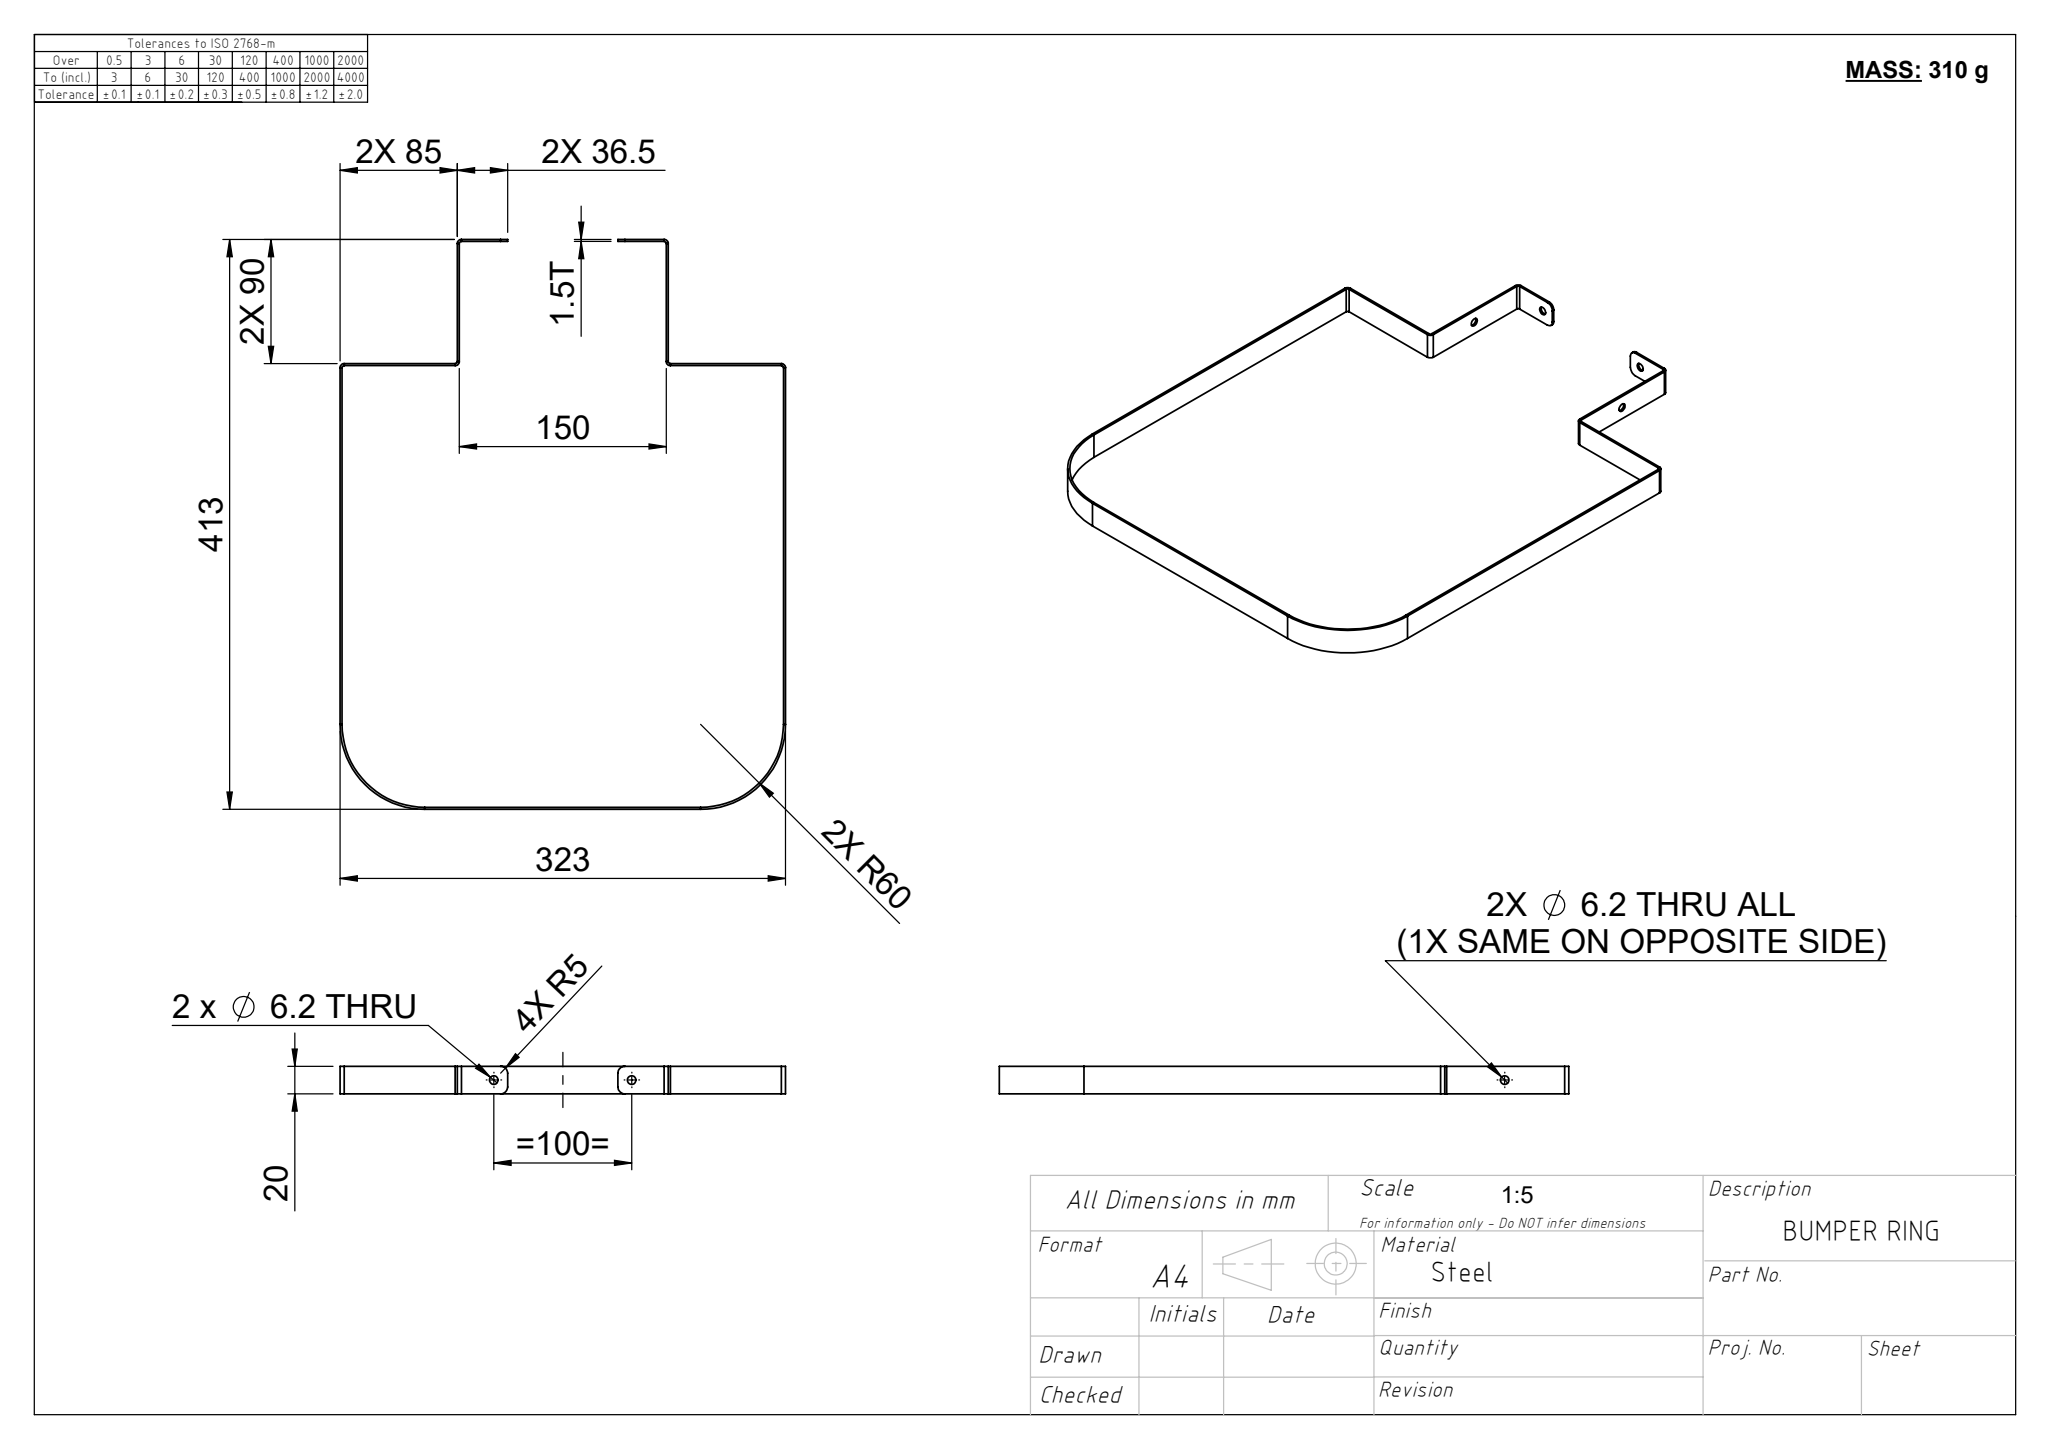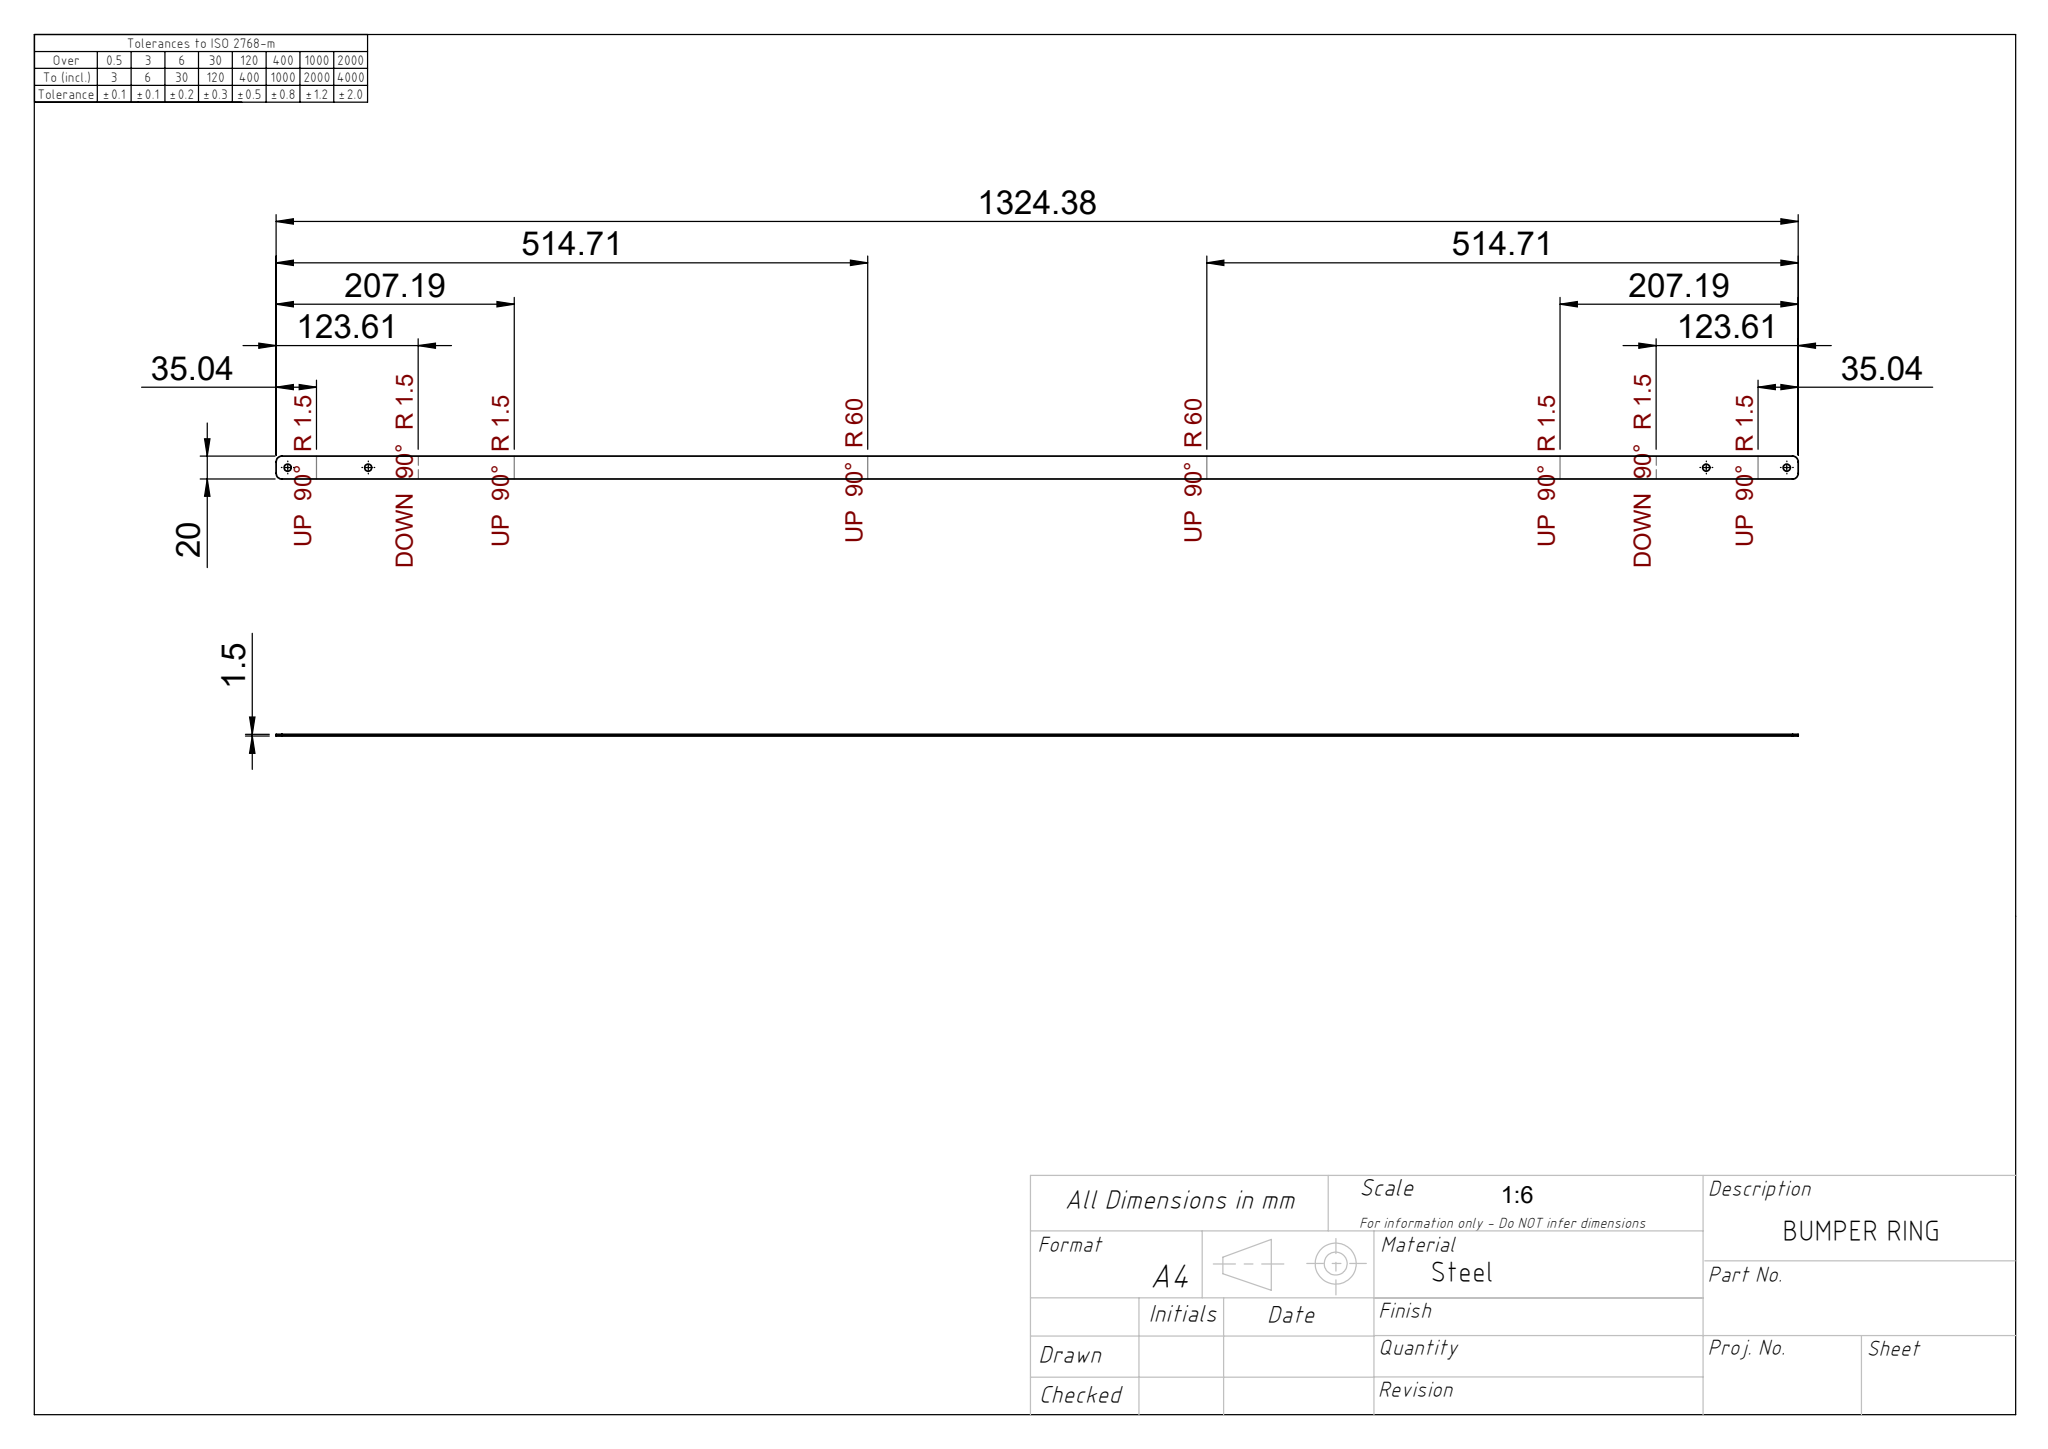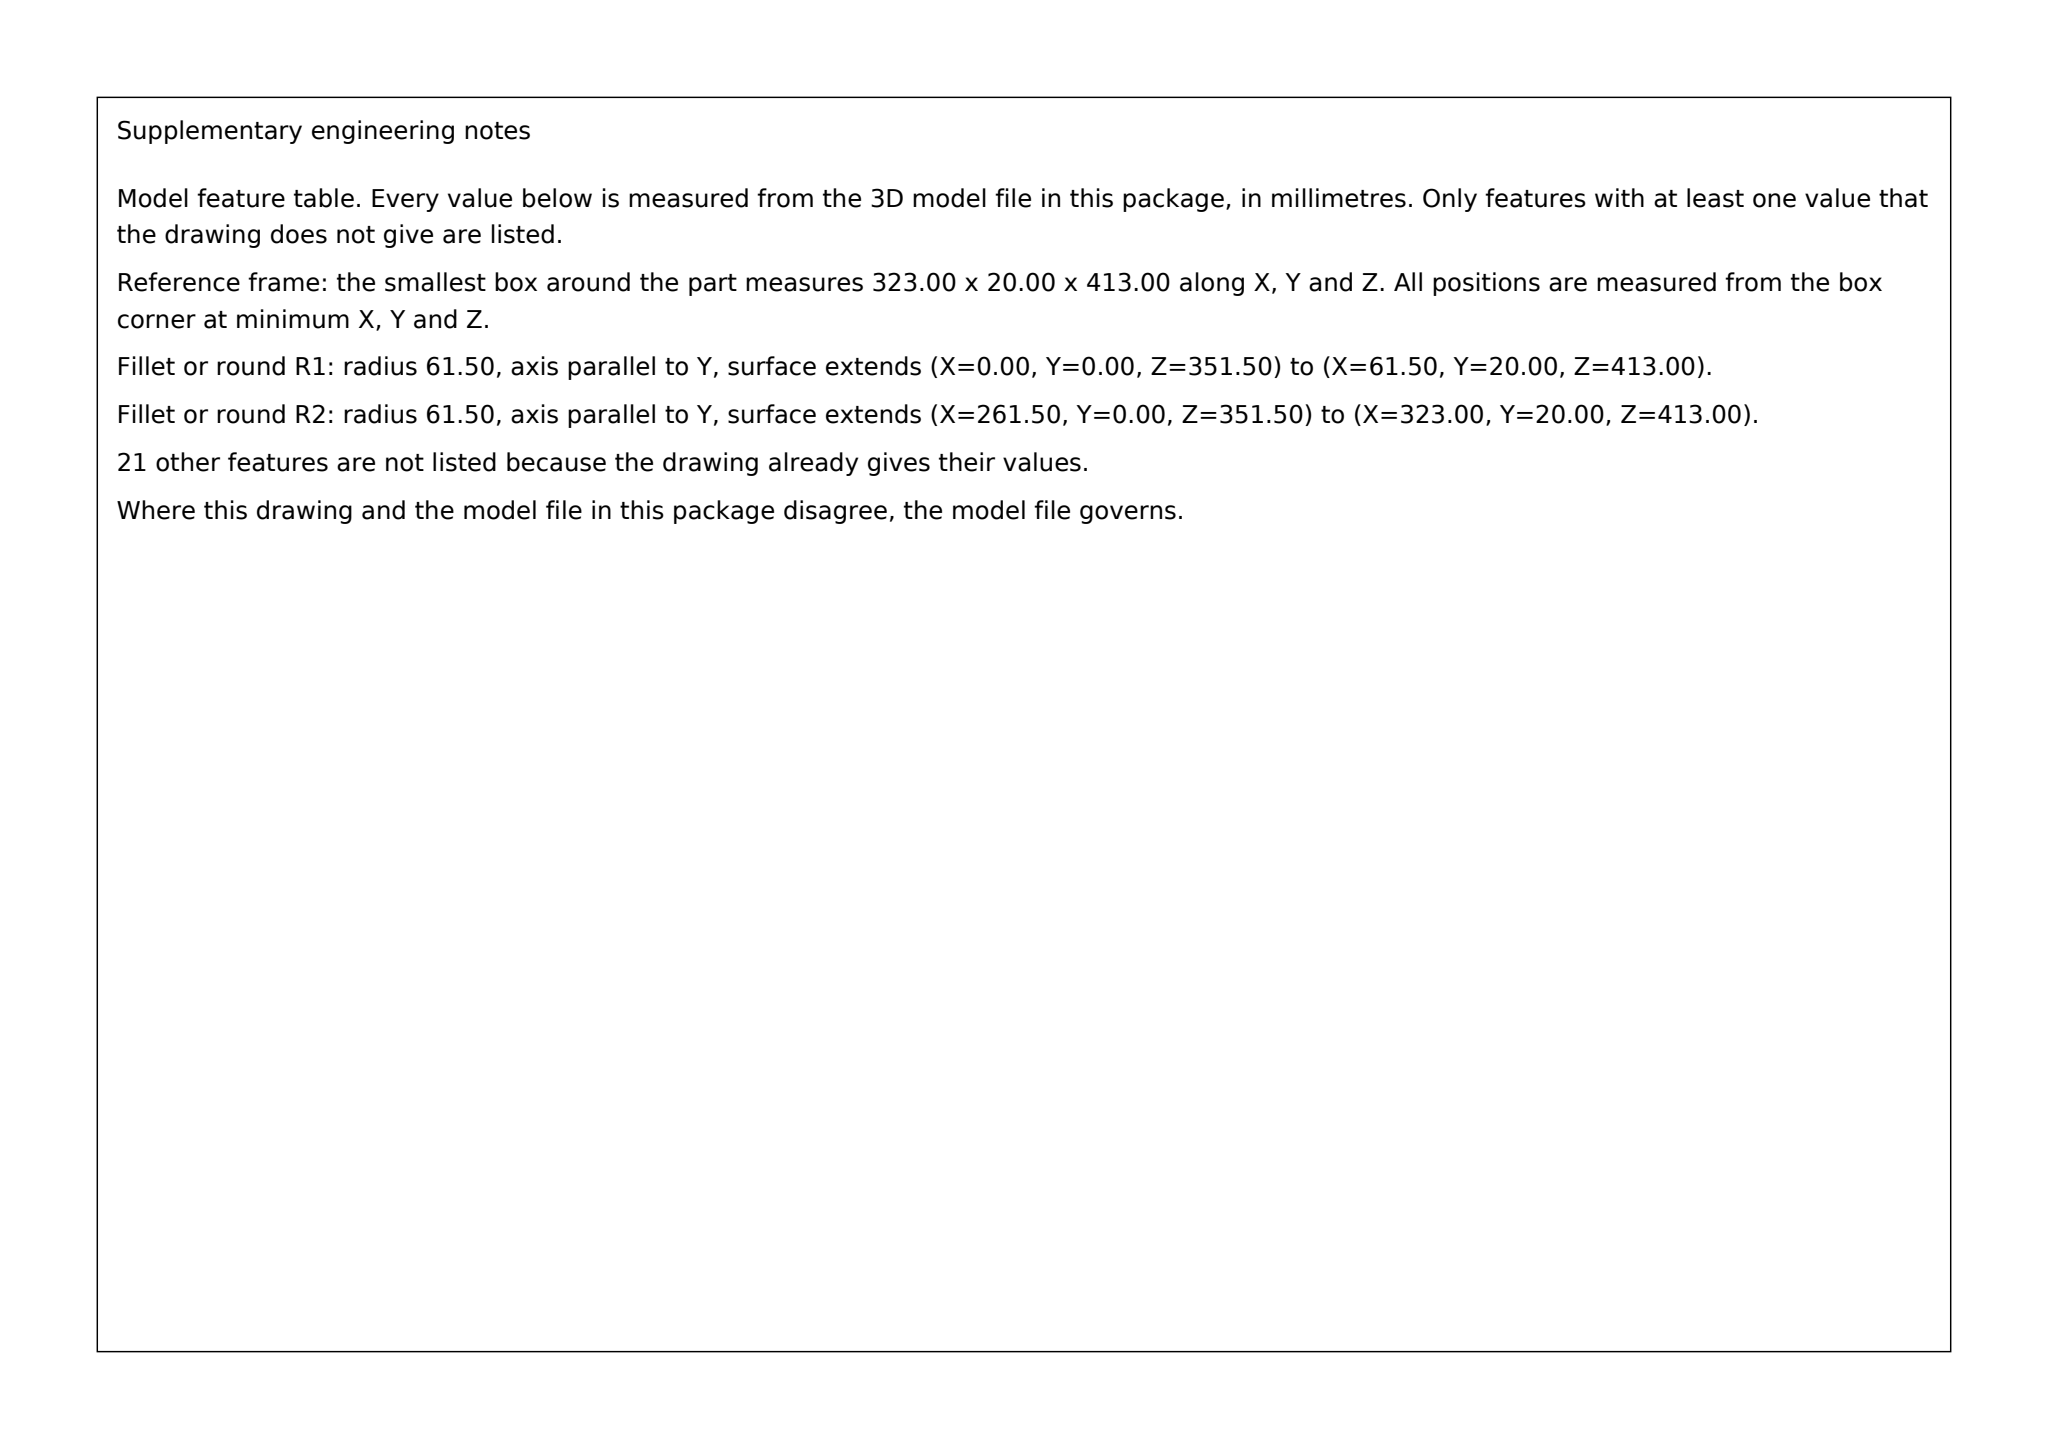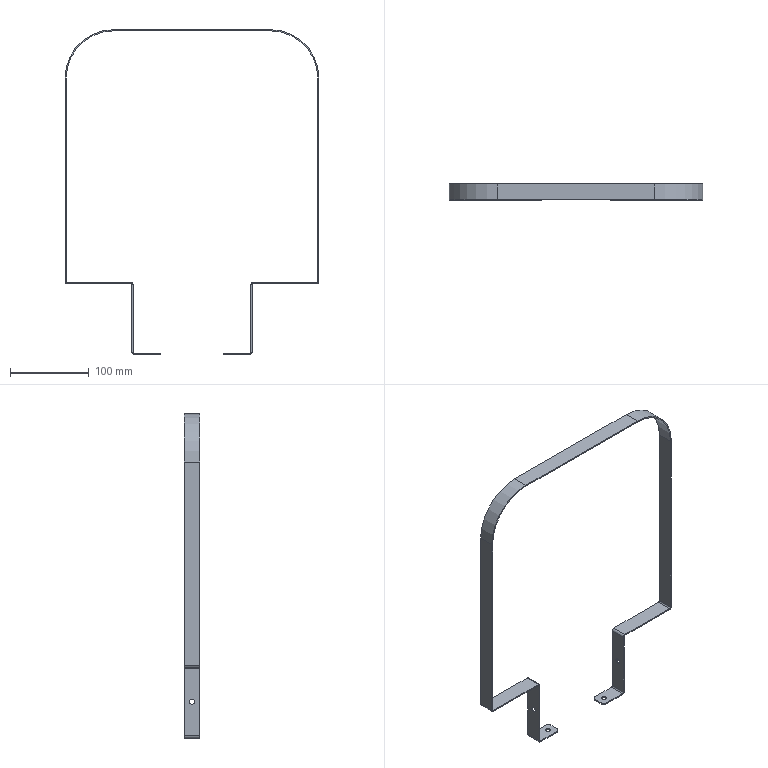Part | SolidWorks | mm | 1 solid | 82 faces | box 323 x 20 x 413 mm | volume 39628 mm3 | plane 54 | cylinder 28 | commonest cylinder face diameters 6.2 x8 3 x6 6 x6 10 x4 120 x2 123 x2
Drawing notes:
4X Ø6.2 THRU the 1.5 mm vertical walls (hole axis parallel to the 323 mm width direction); hole centres 46.5 mm from the bottom outer face of the part, measured in the 413 mm direction. | from the solid: cylinders: [6.2, axis "x", pos (y=10.0, z=46.5), length 1.5, count 4]
These 4X Ø6.2 side-wall holes are centred across the 20 mm strip width: 10 mm from each 20 mm face (y = 10 of 20). | from the solid: cylinders: [6.2, axis "x", pos_other_axes y=10.0, bbox_xyz y = 20.0]
Side-wall Ø6.2 hole set = 4 places total, one in each 1.5 mm wall (walls at x = 0-1.5, 85-86.5, 236.5-238, 321.5-323), arranged symmetrically about the part centreline at x = 161.5 of the 323 mm width. | from the solid: axis_planes x: 0.0, 1.5, 85.0, 86.5, 236.5, 238.0, 321.5, 323.0 with 6.2 dia x-axis cylinders count 4
4X Ø6.2 THRU side walls of tabs (one in each of the four 1.5 thk tab side walls), hole axis normal to the wall. | from the solid: cylinders: [6.2, axis "x", pos [null, 10.0, 46.5], length 1.5, count 4
Side-wall Ø6.2 holes: located 46.5 mm from the tab end face (face at z=0, the 2X 90 tab ends) measured along the 413 direction. | from the solid: cylinders 6.2 axis x at z = 46.5; planes z=0 / z=413 give 413 overall
Side-wall Ø6.2 holes: centred on the 20 mm strip width, 10 mm from each 20 mm face. | from the solid: cylinders 6.2 axis x at y = 10.0; planes y=0 and y=20